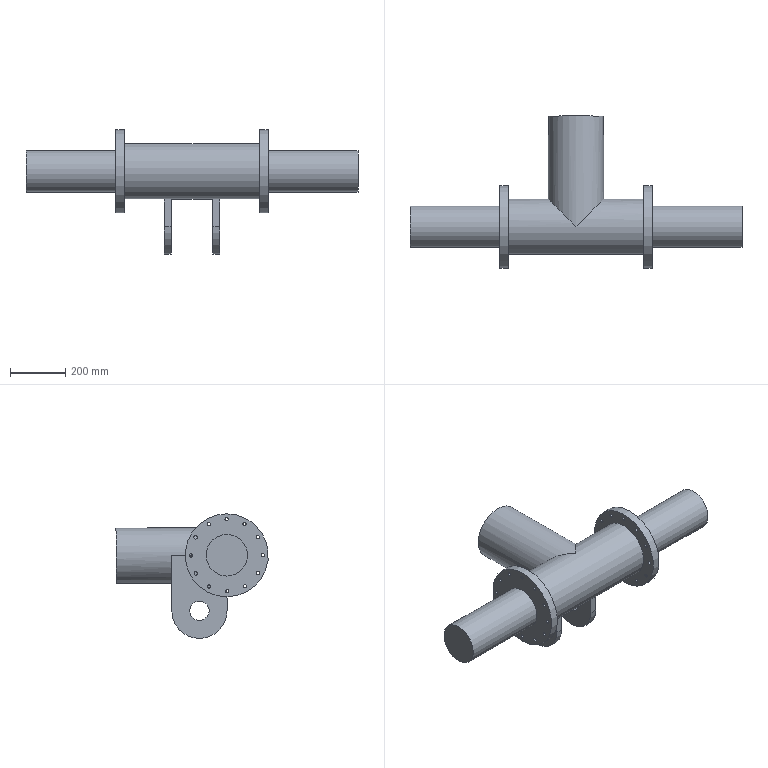Component | NX | AXLE | 1 solid | 52 faces | volume 37121738 mm3 | cylinder 35 | plane 17 | commonest cylinder face diameters 12 x24 200 x4 70 x2 150 x2 300 x2 160 x1